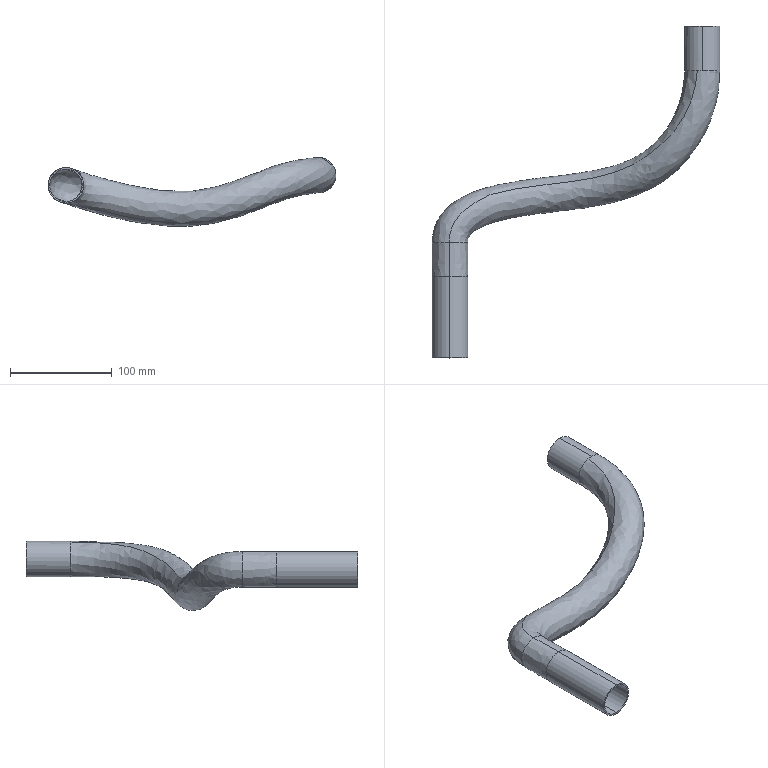Component | SolidWorks | WaterPipe-1 | 1 solid | 16 faces | volume 78860 mm3 | cylinder 8 | spline 6 | plane 2 | commonest cylinder face diameters 35 x4 32 x4